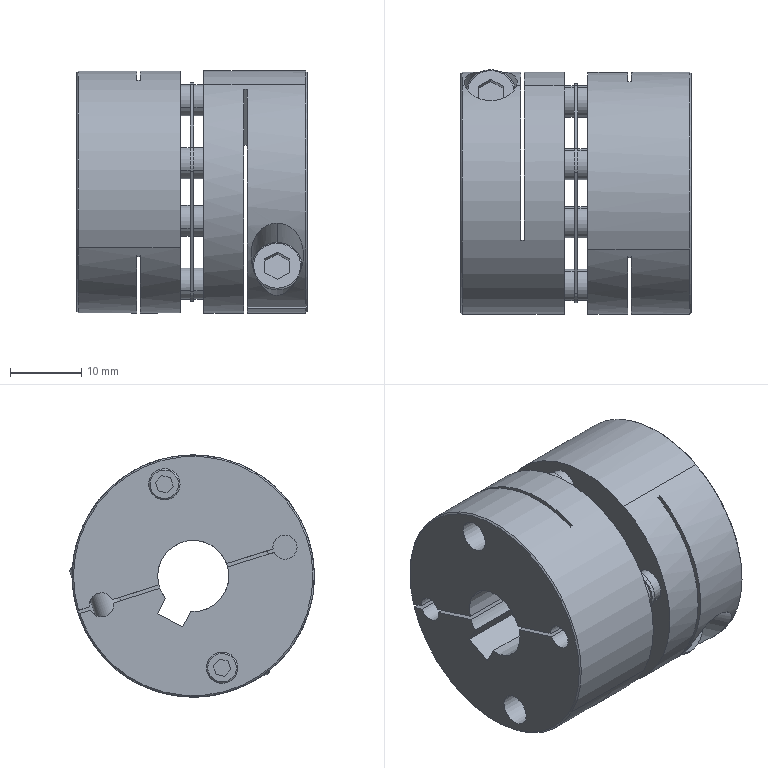Component | SolidWorks | HZ022-D14ToD10(D34x32L)-1 | 1 solid | 209 faces | volume 20839 mm3 | plane 100 | cylinder 86 | cone 23 | commonest cylinder face diameters 4.4 x24 3.4 x14 4.7 x8 4 x8 10 x7 14 x7 34 x6 7.4 x4 | material AL6061